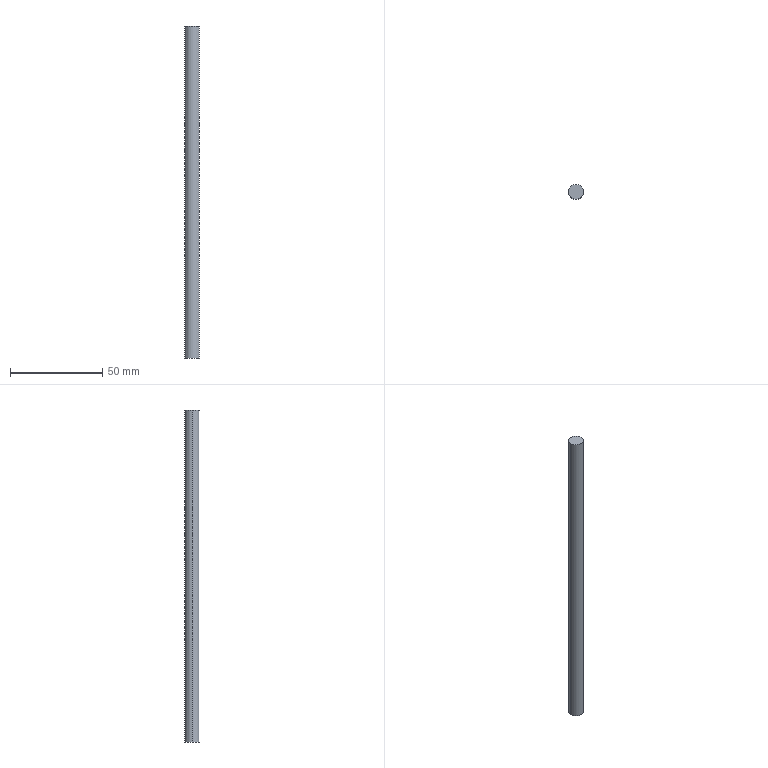Component | SolidWorks | T8LeadScrew-1 | 1 solid | 4 faces | box 8 x 8 x 180 mm | volume 9048 mm3 | cylinder 2 | plane 2 | commonest cylinder face diameters 8 x2
build123d program:
from build123d import *

# Parameters (mm, degrees)
SKETCH1_R           = 4
BOSS_EXTRUDE1_DEPTH = 90


with BuildPart() as part:
    # Sketch1 → Boss-Extrude1 (new, symmetric)
    with BuildSketch(Plane.XY):
        with Locations(Location((0, 0, 0), (0, 0, 180))):
            Circle(SKETCH1_R)
    extrude(amount=BOSS_EXTRUDE1_DEPTH, both=True)


solid = part.part

# Placed as in the assembly
solid = solid.moved(Location((0, 0, 112.5), (0, 0, 0)))
STEP:
#1=COLOUR_RGB('',0.7922,0.8196,0.9333);
#2=FILL_AREA_STYLE_COLOUR('',#1);
#3=FILL_AREA_STYLE('',(#2));
#4=SURFACE_STYLE_FILL_AREA(#3);
#5=SURFACE_SIDE_STYLE('',(#4));
#6=SURFACE_STYLE_USAGE(.BOTH.,#5);
#7=PRESENTATION_STYLE_ASSIGNMENT((#6));
#8=CARTESIAN_POINT('',(-0.1575,0.,7.972));
#9=VERTEX_POINT('',#8);
#10=CARTESIAN_POINT('',(0.1575,0.,7.972));
#11=VERTEX_POINT('',#10);
#12=CARTESIAN_POINT('',(-0.,0.,7.972));
#13=DIRECTION('',(-0.,0.,1.));
#14=DIRECTION('',(-1.,0.,0.));
#15=AXIS2_PLACEMENT_3D('',#12,#13,#14);
#16=CIRCLE('',#15,0.1575);
#17=EDGE_CURVE('',#9,#11,#16,.T.);
#18=ORIENTED_EDGE('',*,*,#17,.F.);
#19=CARTESIAN_POINT('',(-0.1575,0.,0.8858));
#20=VERTEX_POINT('',#19);
#21=CARTESIAN_POINT('',(-0.1575,0.,7.972));
#22=DIRECTION('',(0.,-0.,-1.));
#23=VECTOR('',#22,39.37);
#24=LINE('',#21,#23);
#25=EDGE_CURVE('',#9,#20,#24,.T.);
#26=ORIENTED_EDGE('',*,*,#25,.T.);
#27=CARTESIAN_POINT('',(0.1575,0.,0.8858));
#28=VERTEX_POINT('',#27);
#29=CARTESIAN_POINT('',(-0.,0.,0.8858));
#30=DIRECTION('',(-0.,0.,1.));
#31=DIRECTION('',(-1.,0.,0.));
#32=AXIS2_PLACEMENT_3D('',#29,#30,#31);
#33=CIRCLE('',#32,0.1575);
#34=EDGE_CURVE('',#20,#28,#33,.T.);
#35=ORIENTED_EDGE('',*,*,#34,.T.);
#36=CARTESIAN_POINT('',(0.1575,0.,7.972));
#37=DIRECTION('',(0.,-0.,-1.));
#38=VECTOR('',#37,39.37);
#39=LINE('',#36,#38);
#40=EDGE_CURVE('',#11,#28,#39,.T.);
#41=ORIENTED_EDGE('',*,*,#40,.F.);
#42=EDGE_LOOP('',(#18,#26,#35,#41));
#43=FACE_OUTER_BOUND('',#42,.T.);
#44=CARTESIAN_POINT('',(-0.,0.,7.972));
#45=DIRECTION('',(0.,-0.,-1.));
#46=DIRECTION('',(1.,-0.,0.));
#47=AXIS2_PLACEMENT_3D('',#44,#45,#46);
#48=CYLINDRICAL_SURFACE('',#47,0.1575);
#49=ADVANCED_FACE('',(#43),#48,.T.);
#50=ORIENTED_EDGE('',*,*,#25,.F.);
#51=CARTESIAN_POINT('',(-0.,0.,7.972));
#52=DIRECTION('',(-0.,0.,1.));
#53=DIRECTION('',(-1.,0.,0.));
#54=AXIS2_PLACEMENT_3D('',#51,#52,#53);
#55=CIRCLE('',#54,0.1575);
#56=EDGE_CURVE('',#11,#9,#55,.T.);
#57=ORIENTED_EDGE('',*,*,#56,.F.);
#58=ORIENTED_EDGE('',*,*,#40,.T.);
#59=CARTESIAN_POINT('',(-0.,0.,0.8858));
#60=DIRECTION('',(-0.,0.,1.));
#61=DIRECTION('',(-1.,0.,0.));
#62=AXIS2_PLACEMENT_3D('',#59,#60,#61);
#63=CIRCLE('',#62,0.1575);
#64=EDGE_CURVE('',#28,#20,#63,.T.);
#65=ORIENTED_EDGE('',*,*,#64,.T.);
#66=EDGE_LOOP('',(#50,#57,#58,#65));
#67=FACE_OUTER_BOUND('',#66,.T.);
#68=CARTESIAN_POINT('',(-0.,0.,7.972));
#69=DIRECTION('',(0.,-0.,-1.));
#70=DIRECTION('',(1.,-0.,0.));
#71=AXIS2_PLACEMENT_3D('',#68,#69,#70);
#72=CYLINDRICAL_SURFACE('',#71,0.1575);
#73=ADVANCED_FACE('',(#67),#72,.T.);
#74=ORIENTED_EDGE('',*,*,#56,.T.);
#75=ORIENTED_EDGE('',*,*,#17,.T.);
#76=EDGE_LOOP('',(#74,#75));
#77=FACE_OUTER_BOUND('',#76,.T.);
#78=CARTESIAN_POINT('',(-0.,0.,7.972));
#79=DIRECTION('',(-0.,0.,1.));
#80=DIRECTION('',(-1.,0.,-0.));
#81=AXIS2_PLACEMENT_3D('',#78,#79,#80);
#82=PLANE('',#81);
#83=ADVANCED_FACE('',(#77),#82,.T.);
#84=ORIENTED_EDGE('',*,*,#64,.F.);
#85=ORIENTED_EDGE('',*,*,#34,.F.);
#86=EDGE_LOOP('',(#84,#85));
#87=FACE_OUTER_BOUND('',#86,.T.);
#88=CARTESIAN_POINT('',(-0.,0.,0.8858));
#89=DIRECTION('',(-0.,0.,1.));
#90=DIRECTION('',(-1.,0.,-0.));
#91=AXIS2_PLACEMENT_3D('',#88,#89,#90);
#92=PLANE('',#91);
#93=ADVANCED_FACE('',(#87),#92,.F.);
#94=CLOSED_SHELL('',(#49,#73,#83,#93));
#95=MANIFOLD_SOLID_BREP('',#94);
#96=STYLED_ITEM('',(#7),#95);
#97=(LENGTH_UNIT()NAMED_UNIT(*)SI_UNIT($,.METRE.));
#98=LENGTH_MEASURE_WITH_UNIT(LENGTH_MEASURE(0.0254),#97);
#99=DIMENSIONAL_EXPONENTS(1.,0.,0.,0.,0.,0.,0.);
#100=(CONVERSION_BASED_UNIT('',#98)LENGTH_UNIT()NAMED_UNIT(#99));
#101=UNCERTAINTY_MEASURE_WITH_UNIT(LENGTH_MEASURE(0.00001),#100,'','');
#102=(NAMED_UNIT(*)PLANE_ANGLE_UNIT()SI_UNIT($,.RADIAN.));
#103=(NAMED_UNIT(*)SI_UNIT($,.STERADIAN.)SOLID_ANGLE_UNIT());
#104=(GEOMETRIC_REPRESENTATION_CONTEXT(3)GLOBAL_UNCERTAINTY_ASSIGNED_CONTEXT((#101))GLOBAL_UNIT_ASSIGNED_CONTEXT((#100,#102,#103))REPRESENTATION_CONTEXT('',''));
#105=MECHANICAL_DESIGN_GEOMETRIC_PRESENTATION_REPRESENTATION('',(#96),#104);
#106=CARTESIAN_POINT('',(0.,0.,0.));
#107=DIRECTION('',(0.,0.,1.));
#108=DIRECTION('',(1.,0.,0.));
#109=AXIS2_PLACEMENT_3D('',#106,#107,#108);
#110=(LENGTH_UNIT()NAMED_UNIT(*)SI_UNIT($,.METRE.));
#111=LENGTH_MEASURE_WITH_UNIT(LENGTH_MEASURE(0.0254),#110);
#112=DIMENSIONAL_EXPONENTS(1.,0.,0.,0.,0.,0.,0.);
#113=(CONVERSION_BASED_UNIT('',#111)LENGTH_UNIT()NAMED_UNIT(#112));
#114=UNCERTAINTY_MEASURE_WITH_UNIT(LENGTH_MEASURE(0.00001),#113,'','');
#115=(NAMED_UNIT(*)PLANE_ANGLE_UNIT()SI_UNIT($,.RADIAN.));
#116=(NAMED_UNIT(*)SI_UNIT($,.STERADIAN.)SOLID_ANGLE_UNIT());
#117=(GEOMETRIC_REPRESENTATION_CONTEXT(3)GLOBAL_UNCERTAINTY_ASSIGNED_CONTEXT((#114))GLOBAL_UNIT_ASSIGNED_CONTEXT((#113,#115,#116))REPRESENTATION_CONTEXT('',''));
#118=ADVANCED_BREP_SHAPE_REPRESENTATION('',(#95,#109),#117);
#119=PRESENTATION_LAYER_ASSIGNMENT('','',(#96));